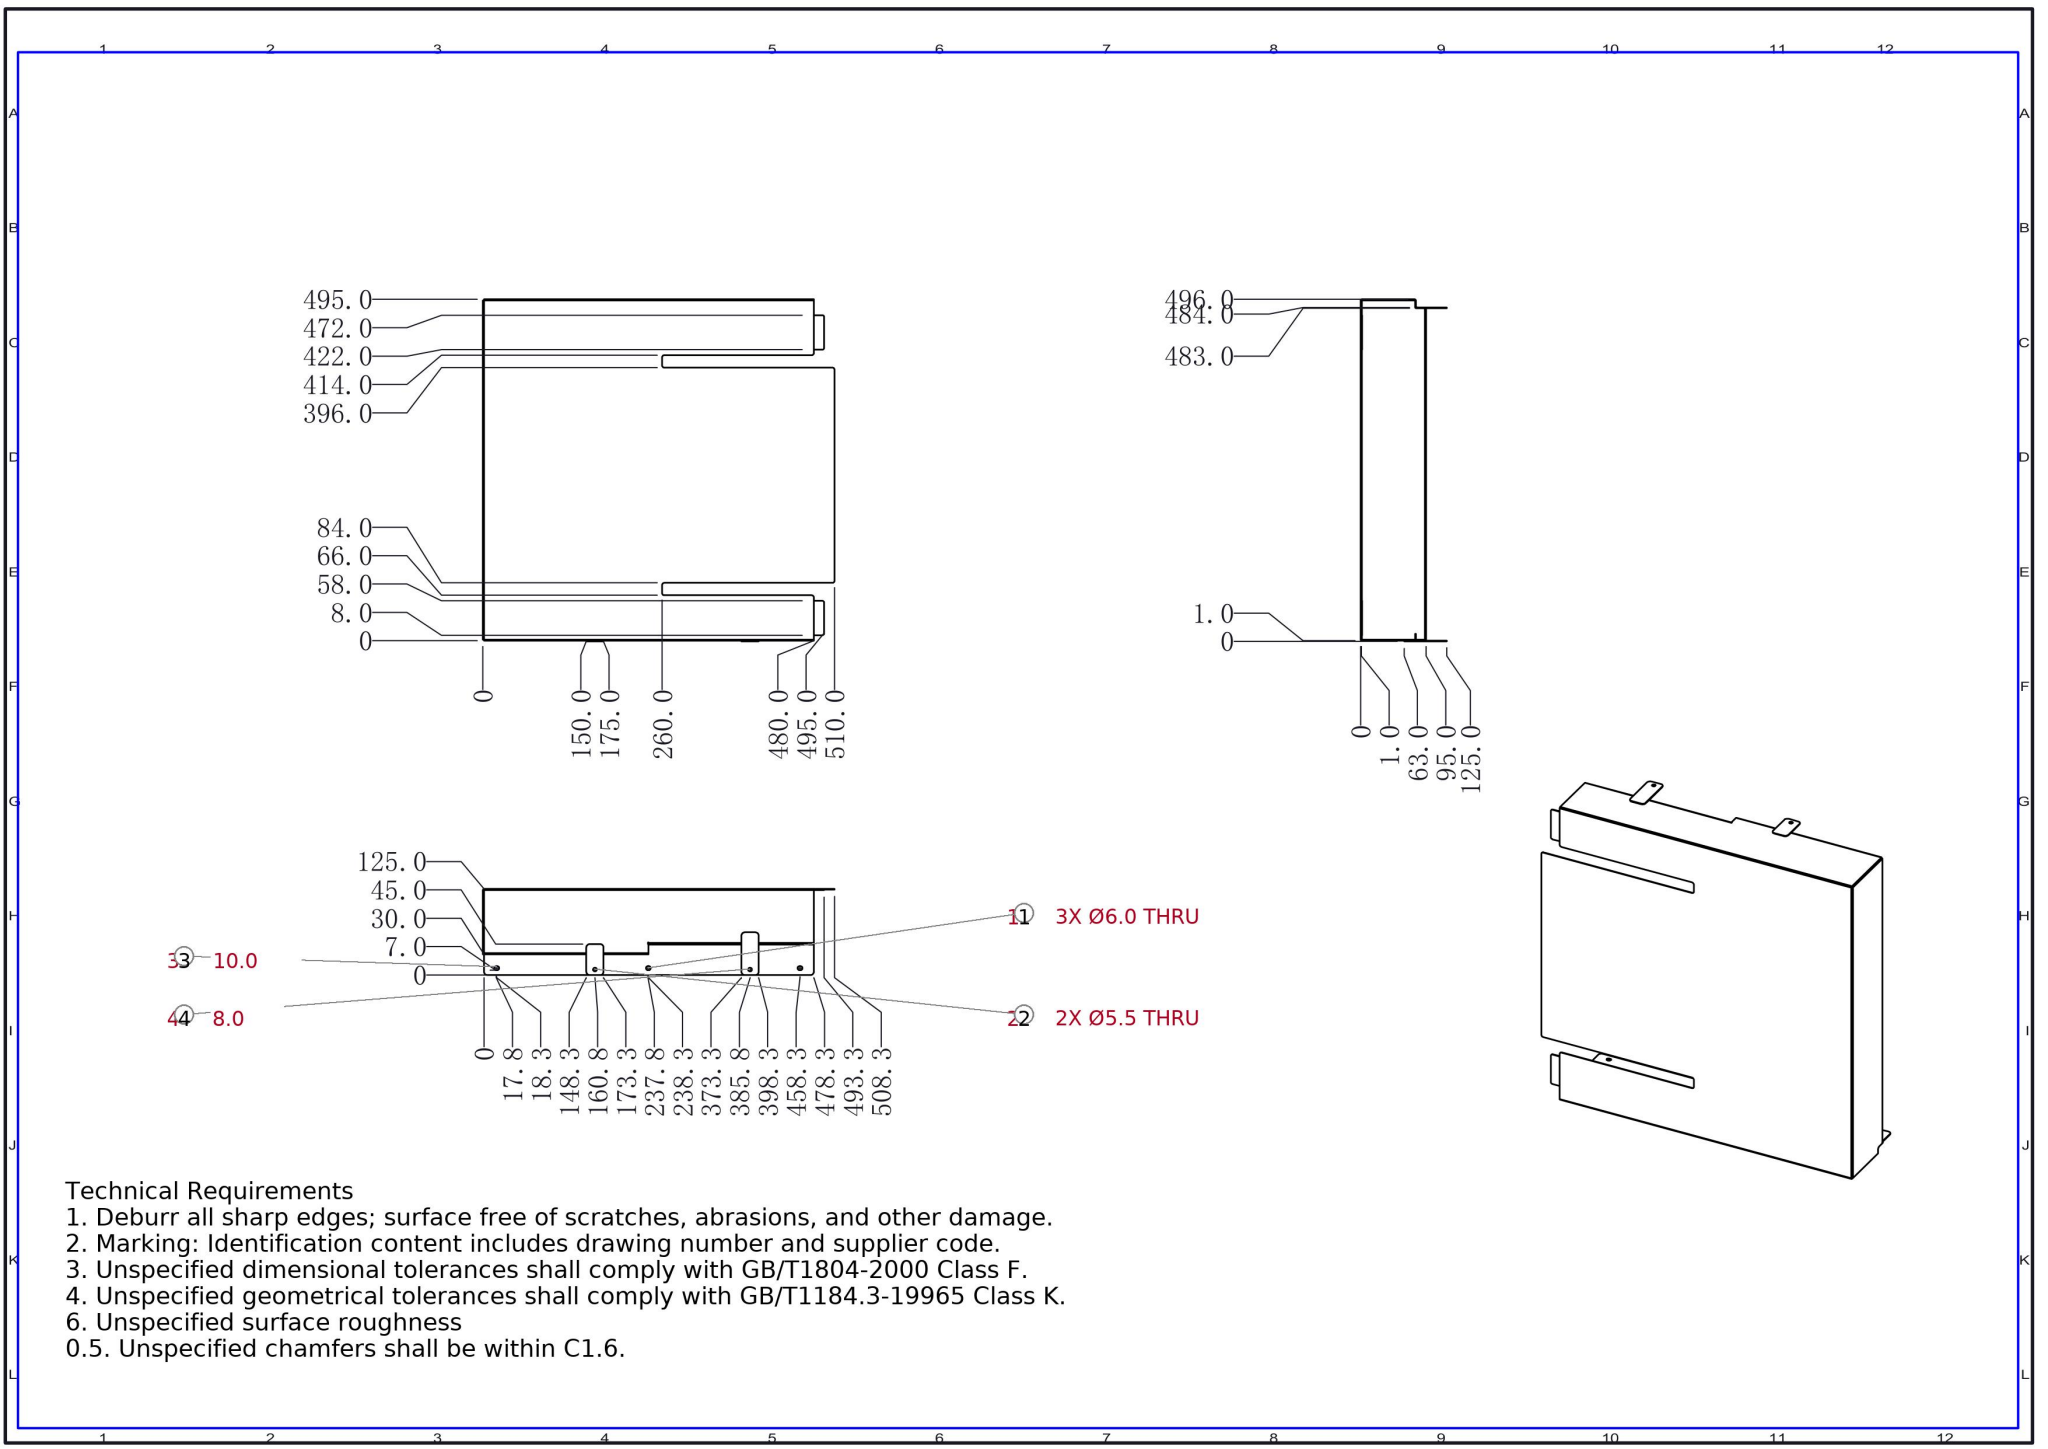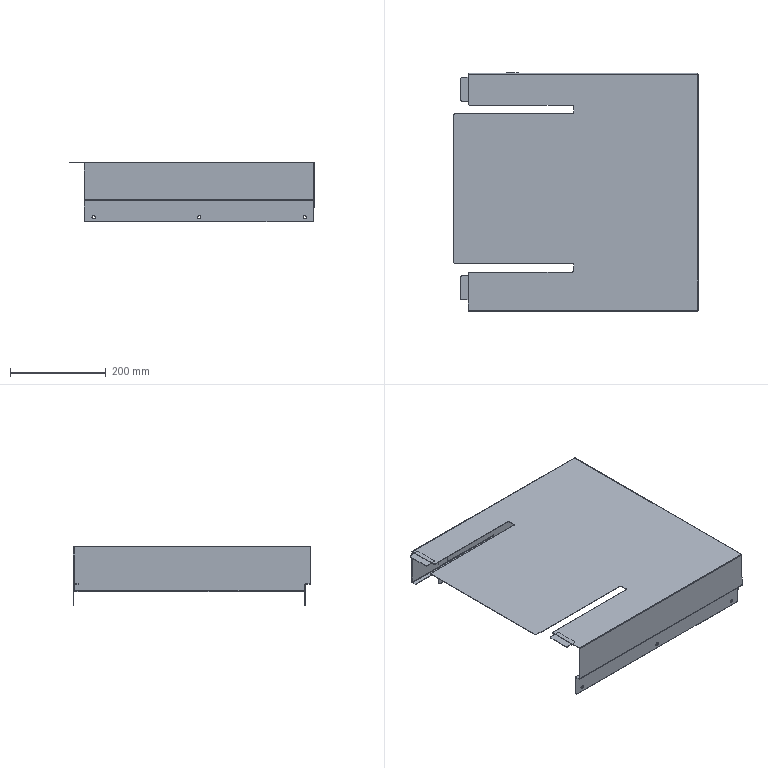Part | SolidWorks | mm | 1 solid | 157 faces | box 510 x 496 x 125 mm | volume 403203 mm3 | plane 98 | cylinder 53 | spline 6 | commonest cylinder face diameters 6 x23 10 x10 3.473 x8 1.473 x8 5.5 x4